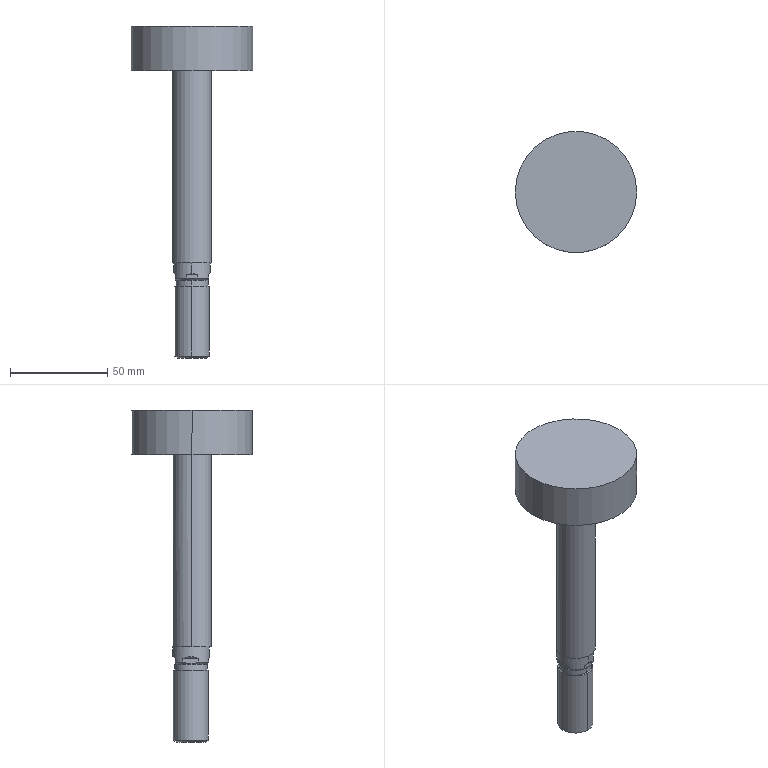Component | SolidWorks | NewCurveBenderSDAT63x45x45Cylinder-DoubleWheel-1_NewTypeCurveBenderSDATS-63x45x45-B_4545r-DoubleWheel-1 | 1 solid | 27 faces | box 62.5 x 62.5 x 171 mm | volume 114115 mm3 | plane 14 | cylinder 10 | cone 3 | commonest cylinder face diameters 18.866 x2 16.666 x2 18 x2 62.5 x2 20 x2
build123d program:
from build123d import *

# Parameters (mm, degrees)
CUT_EXTRUDE1_DEPTH      = 17
CUT_EXTRUDE1_DEPTH_BACK = 17
CUT_EXTRUDE2_DEPTH      = 17
CUT_EXTRUDE2_DEPTH_BACK = 17


with BuildPart() as part:
    # Sketch1 → Revolve1 (revolve)
    with BuildSketch(Plane.XY, mode=Mode.PRIVATE) as revolve1_sk:
        Polygon((0, 0), (0, 10), (99, 10), (99, 31.25), (122, 31.25), (122, 0), align=None)
    revolve(revolve1_sk.sketch.rotate(Axis((122, 0, 0), (-1, 0, 0)), 270), axis=Axis((122, 0, 0), (-1, 0, 0)))

    # Sketch2 → Revolve2 (revolve)
    with BuildSketch(Plane.XY, mode=Mode.PRIVATE) as revolve2_sk:
        Polygon((-49, 0.5669), (-49, 8.08), (-48.001, 9.567), (-12, 9.567), (-12, 8.9), (-9, 8.9), (-7.9, 10), (0, 10), (0, 0.5669), align=None)
    revolve(revolve2_sk.sketch.rotate(Axis((0, 0.5669, 0), (-1, 0, 0)), 180), axis=Axis((0, 0.5669, 0), (-1, 0, 0)))

    # Sketch3 → Cut-Extrude1 (cut, two sides: drawn at the far end of the back side and taken through both)
    with BuildSketch(Plane(origin=(0, 0, 0), x_dir=(1, 0, 0), z_dir=(0, 1, 0)).offset(-CUT_EXTRUDE1_DEPTH_BACK)):
        Polygon((-59.877, -13.5), (-1, -13.5), (-6, -8.5), (-9, -8.5), (-9, -11), (-51.624, -11), (-51.624, 11), (-9, 11), (-9, 8.5), (-6, 8.5), (-1, 13.5), (-59.877, 13.5), align=None)
    extrude(amount=CUT_EXTRUDE1_DEPTH + CUT_EXTRUDE1_DEPTH_BACK, mode=Mode.SUBTRACT)

    # Sketch4 → Cut-Extrude2 (cut, two sides: drawn at the far end of the back side and taken through both)
    with BuildSketch(Plane.XY.offset(-CUT_EXTRUDE2_DEPTH_BACK)):
        Polygon((-59.696, -13.5), (-1, -13.5), (-6, -8.5), (-9, -8.5), (-9, -11), (-52.973, -11), (-52.973, 11), (-9, 11), (-9, 8.5), (-6, 8.5), (-1, 13.5), (-59.696, 13.5), align=None)
    extrude(amount=CUT_EXTRUDE2_DEPTH + CUT_EXTRUDE2_DEPTH_BACK, mode=Mode.SUBTRACT)


solid = part.part

# Placed as in the assembly
solid = solid.moved(Location((0, 47, 237.459), (0, -90, 0)))